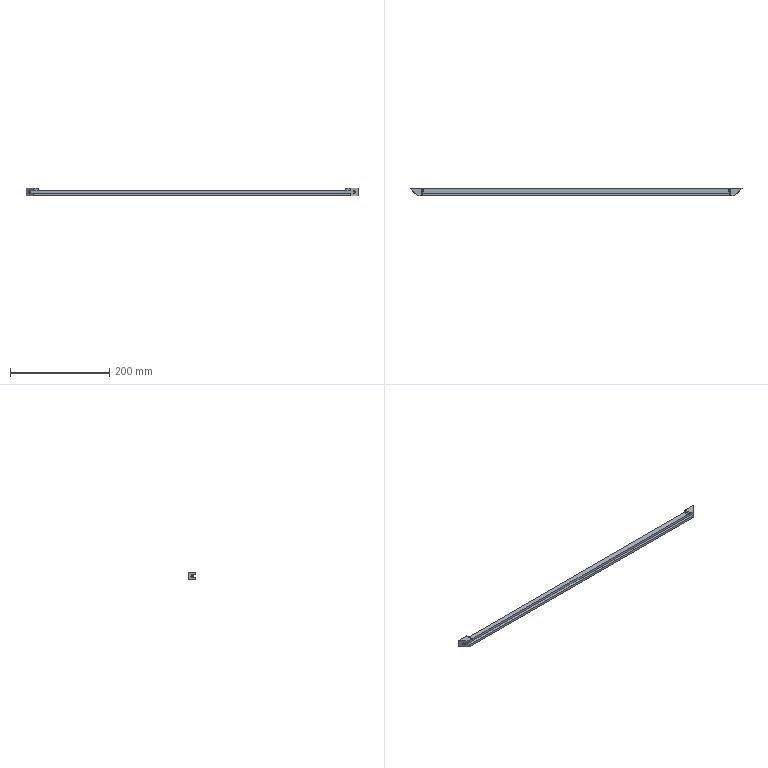Component | SolidWorks | AUTO-SpinDryWashing-01-03000006-1 | 1 solid | 30 faces | box 670 x 15 x 15 mm | volume 84011 mm3 | plane 18 | cylinder 12 | commonest cylinder face diameters 4.5 x4 8 x4 4 x4 | material AISI 304
STEP:
#1=CARTESIAN_POINT('',(-12.973,31.202,2.264));
#2=VERTEX_POINT('',#1);
#3=CARTESIAN_POINT('',(-12.848,31.076,2.264));
#4=VERTEX_POINT('',#3);
#5=CARTESIAN_POINT('',(-12.911,31.139,2.264));
#6=DIRECTION('',(-0.7071,-0.7071,-0.));
#7=DIRECTION('',(0.7071,-0.7071,0.));
#8=AXIS2_PLACEMENT_3D('',#5,#6,#7);
#9=CIRCLE('',#8,0.08858);
#10=EDGE_CURVE('',#2,#4,#9,.T.);
#11=ORIENTED_EDGE('',*,*,#10,.T.);
#12=CARTESIAN_POINT('',(-12.737,31.188,2.264));
#13=VERTEX_POINT('',#12);
#14=CARTESIAN_POINT('',(-12.458,31.466,2.264));
#15=DIRECTION('',(0.7071,0.7071,0.));
#16=VECTOR('',#15,39.37);
#17=LINE('',#14,#16);
#18=EDGE_CURVE('',#4,#13,#17,.T.);
#19=ORIENTED_EDGE('',*,*,#18,.T.);
#20=CARTESIAN_POINT('',(-12.862,31.313,2.264));
#21=VERTEX_POINT('',#20);
#22=CARTESIAN_POINT('',(-12.799,31.25,2.264));
#23=DIRECTION('',(0.7071,0.7071,0.));
#24=DIRECTION('',(-0.7071,0.7071,0.));
#25=AXIS2_PLACEMENT_3D('',#22,#23,#24);
#26=CIRCLE('',#25,0.08858);
#27=EDGE_CURVE('',#13,#21,#26,.T.);
#28=ORIENTED_EDGE('',*,*,#27,.T.);
#29=CARTESIAN_POINT('',(-12.583,31.591,2.264));
#30=DIRECTION('',(0.7071,0.7071,0.));
#31=VECTOR('',#30,39.37);
#32=LINE('',#29,#31);
#33=EDGE_CURVE('',#2,#21,#32,.T.);
#34=ORIENTED_EDGE('',*,*,#33,.F.);
#35=EDGE_LOOP('',(#11,#19,#28,#34));
#36=FACE_OUTER_BOUND('',#35,.T.);
#37=CARTESIAN_POINT('',(-12.521,31.529,2.264));
#38=DIRECTION('',(0.7071,0.7071,0.));
#39=DIRECTION('',(-0.7071,0.7071,0.));
#40=AXIS2_PLACEMENT_3D('',#37,#38,#39);
#41=CYLINDRICAL_SURFACE('',#40,0.08858);
#42=ADVANCED_FACE('',(#36),#41,.F.);
#43=CARTESIAN_POINT('',(-12.688,31.139,2.264));
#44=VERTEX_POINT('',#43);
#45=CARTESIAN_POINT('',(-12.911,31.362,2.264));
#46=VERTEX_POINT('',#45);
#47=CARTESIAN_POINT('',(-12.799,31.25,2.264));
#48=DIRECTION('',(0.7071,0.7071,0.));
#49=DIRECTION('',(-0.7071,0.7071,0.));
#50=AXIS2_PLACEMENT_3D('',#47,#48,#49);
#51=CIRCLE('',#50,0.1575);
#52=EDGE_CURVE('',#44,#46,#51,.T.);
#53=ORIENTED_EDGE('',*,*,#52,.F.);
#54=CARTESIAN_POINT('',(-12.409,31.417,2.264));
#55=VERTEX_POINT('',#54);
#56=CARTESIAN_POINT('',(-12.409,31.417,2.264));
#57=DIRECTION('',(0.7071,0.7071,0.));
#58=VECTOR('',#57,39.37);
#59=LINE('',#56,#58);
#60=EDGE_CURVE('',#44,#55,#59,.T.);
#61=ORIENTED_EDGE('',*,*,#60,.T.);
#62=CARTESIAN_POINT('',(-12.855,31.417,2.264));
#63=VERTEX_POINT('',#62);
#64=CARTESIAN_POINT('',(-12.855,31.417,2.264));
#65=CARTESIAN_POINT('',(-12.855,31.417,1.949));
#66=CARTESIAN_POINT('',(-12.409,31.417,1.949));
#67=CARTESIAN_POINT('',(-12.409,31.417,2.264));
#68=(BOUNDED_CURVE()B_SPLINE_CURVE(3,(#64,#65,#66,#67),.UNSPECIFIED.,.F.,.T.)B_SPLINE_CURVE_WITH_KNOTS((4,4),(3.142,6.283),.UNSPECIFIED.)CURVE()GEOMETRIC_REPRESENTATION_ITEM()RATIONAL_B_SPLINE_CURVE((1.,0.3333,0.3333,1.))REPRESENTATION_ITEM(''));
#69=EDGE_CURVE('',#63,#55,#68,.T.);
#70=ORIENTED_EDGE('',*,*,#69,.F.);
#71=CARTESIAN_POINT('',(-12.632,31.64,2.264));
#72=DIRECTION('',(0.7071,0.7071,0.));
#73=VECTOR('',#72,39.37);
#74=LINE('',#71,#73);
#75=EDGE_CURVE('',#46,#63,#74,.T.);
#76=ORIENTED_EDGE('',*,*,#75,.F.);
#77=EDGE_LOOP('',(#53,#61,#70,#76));
#78=FACE_OUTER_BOUND('',#77,.T.);
#79=CARTESIAN_POINT('',(-12.521,31.529,2.264));
#80=DIRECTION('',(0.7071,0.7071,0.));
#81=DIRECTION('',(-0.7071,0.7071,0.));
#82=AXIS2_PLACEMENT_3D('',#79,#80,#81);
#83=CYLINDRICAL_SURFACE('',#82,0.1575);
#84=ADVANCED_FACE('',(#78),#83,.F.);
#85=CARTESIAN_POINT('',(12.973,31.202,2.264));
#86=VERTEX_POINT('',#85);
#87=CARTESIAN_POINT('',(12.848,31.076,2.264));
#88=VERTEX_POINT('',#87);
#89=CARTESIAN_POINT('',(12.911,31.139,2.264));
#90=DIRECTION('',(-0.7071,0.7071,-0.));
#91=DIRECTION('',(-0.7071,-0.7071,0.));
#92=AXIS2_PLACEMENT_3D('',#89,#90,#91);
#93=CIRCLE('',#92,0.08858);
#94=EDGE_CURVE('',#86,#88,#93,.T.);
#95=ORIENTED_EDGE('',*,*,#94,.F.);
#96=CARTESIAN_POINT('',(12.862,31.313,2.264));
#97=VERTEX_POINT('',#96);
#98=CARTESIAN_POINT('',(12.583,31.591,2.264));
#99=DIRECTION('',(-0.7071,0.7071,-0.));
#100=VECTOR('',#99,39.37);
#101=LINE('',#98,#100);
#102=EDGE_CURVE('',#86,#97,#101,.T.);
#103=ORIENTED_EDGE('',*,*,#102,.T.);
#104=CARTESIAN_POINT('',(12.737,31.188,2.264));
#105=VERTEX_POINT('',#104);
#106=CARTESIAN_POINT('',(12.799,31.25,2.264));
#107=DIRECTION('',(-0.7071,0.7071,-0.));
#108=DIRECTION('',(-0.7071,-0.7071,0.));
#109=AXIS2_PLACEMENT_3D('',#106,#107,#108);
#110=CIRCLE('',#109,0.08858);
#111=EDGE_CURVE('',#97,#105,#110,.T.);
#112=ORIENTED_EDGE('',*,*,#111,.T.);
#113=CARTESIAN_POINT('',(12.458,31.466,2.264));
#114=DIRECTION('',(-0.7071,0.7071,-0.));
#115=VECTOR('',#114,39.37);
#116=LINE('',#113,#115);
#117=EDGE_CURVE('',#88,#105,#116,.T.);
#118=ORIENTED_EDGE('',*,*,#117,.F.);
#119=EDGE_LOOP('',(#95,#103,#112,#118));
#120=FACE_OUTER_BOUND('',#119,.T.);
#121=CARTESIAN_POINT('',(12.521,31.529,2.264));
#122=DIRECTION('',(-0.7071,0.7071,-0.));
#123=DIRECTION('',(-0.7071,-0.7071,0.));
#124=AXIS2_PLACEMENT_3D('',#121,#122,#123);
#125=CYLINDRICAL_SURFACE('',#124,0.08858);
#126=ADVANCED_FACE('',(#120),#125,.F.);
#127=CARTESIAN_POINT('',(12.911,31.362,2.264));
#128=VERTEX_POINT('',#127);
#129=CARTESIAN_POINT('',(12.688,31.139,2.264));
#130=VERTEX_POINT('',#129);
#131=CARTESIAN_POINT('',(12.799,31.25,2.264));
#132=DIRECTION('',(-0.7071,0.7071,-0.));
#133=DIRECTION('',(-0.7071,-0.7071,0.));
#134=AXIS2_PLACEMENT_3D('',#131,#132,#133);
#135=CIRCLE('',#134,0.1575);
#136=EDGE_CURVE('',#128,#130,#135,.T.);
#137=ORIENTED_EDGE('',*,*,#136,.F.);
#138=CARTESIAN_POINT('',(12.855,31.417,2.264));
#139=VERTEX_POINT('',#138);
#140=CARTESIAN_POINT('',(12.632,31.64,2.264));
#141=DIRECTION('',(-0.7071,0.7071,-0.));
#142=VECTOR('',#141,39.37);
#143=LINE('',#140,#142);
#144=EDGE_CURVE('',#128,#139,#143,.T.);
#145=ORIENTED_EDGE('',*,*,#144,.T.);
#146=CARTESIAN_POINT('',(12.409,31.417,2.264));
#147=VERTEX_POINT('',#146);
#148=CARTESIAN_POINT('',(12.409,31.417,2.264));
#149=CARTESIAN_POINT('',(12.409,31.417,1.949));
#150=CARTESIAN_POINT('',(12.855,31.417,1.949));
#151=CARTESIAN_POINT('',(12.855,31.417,2.264));
#152=(BOUNDED_CURVE()B_SPLINE_CURVE(3,(#148,#149,#150,#151),.UNSPECIFIED.,.F.,.F.)B_SPLINE_CURVE_WITH_KNOTS((4,4),(-0.,3.142),.UNSPECIFIED.)CURVE()GEOMETRIC_REPRESENTATION_ITEM()RATIONAL_B_SPLINE_CURVE((1.,0.3333,0.3333,1.))REPRESENTATION_ITEM(''));
#153=EDGE_CURVE('',#147,#139,#152,.T.);
#154=ORIENTED_EDGE('',*,*,#153,.F.);
#155=CARTESIAN_POINT('',(12.409,31.417,2.264));
#156=DIRECTION('',(-0.7071,0.7071,-0.));
#157=VECTOR('',#156,39.37);
#158=LINE('',#155,#157);
#159=EDGE_CURVE('',#130,#147,#158,.T.);
#160=ORIENTED_EDGE('',*,*,#159,.F.);
#161=EDGE_LOOP('',(#137,#145,#154,#160));
#162=FACE_OUTER_BOUND('',#161,.T.);
#163=CARTESIAN_POINT('',(12.521,31.529,2.264));
#164=DIRECTION('',(-0.7071,0.7071,-0.));
#165=DIRECTION('',(-0.7071,-0.7071,0.));
#166=AXIS2_PLACEMENT_3D('',#163,#164,#165);
#167=CYLINDRICAL_SURFACE('',#166,0.1575);
#168=ADVANCED_FACE('',(#162),#167,.F.);
#169=CARTESIAN_POINT('',(12.598,30.827,2.559));
#170=VERTEX_POINT('',#169);
#171=CARTESIAN_POINT('',(12.283,30.827,2.559));
#172=VERTEX_POINT('',#171);
#173=CARTESIAN_POINT('',(13.189,30.827,2.559));
#174=DIRECTION('',(-1.,0.,-0.));
#175=VECTOR('',#174,39.37);
#176=LINE('',#173,#175);
#177=EDGE_CURVE('',#170,#172,#176,.T.);
#178=ORIENTED_EDGE('',*,*,#177,.T.);
#179=CARTESIAN_POINT('',(12.205,30.827,2.48));
#180=VERTEX_POINT('',#179);
#181=CARTESIAN_POINT('',(12.283,30.827,2.48));
#182=DIRECTION('',(0.,-1.,0.));
#183=DIRECTION('',(1.,0.,0.));
#184=AXIS2_PLACEMENT_3D('',#181,#182,#183);
#185=CIRCLE('',#184,0.07874);
#186=EDGE_CURVE('',#172,#180,#185,.T.);
#187=ORIENTED_EDGE('',*,*,#186,.T.);
#188=CARTESIAN_POINT('',(12.205,30.827,2.362));
#189=VERTEX_POINT('',#188);
#190=CARTESIAN_POINT('',(12.205,30.827,1.969));
#191=DIRECTION('',(-0.,-0.,1.));
#192=VECTOR('',#191,39.37);
#193=LINE('',#190,#192);
#194=EDGE_CURVE('',#189,#180,#193,.T.);
#195=ORIENTED_EDGE('',*,*,#194,.F.);
#196=CARTESIAN_POINT('',(12.598,30.827,2.362));
#197=VERTEX_POINT('',#196);
#198=CARTESIAN_POINT('',(13.189,30.827,2.362));
#199=DIRECTION('',(-1.,0.,-0.));
#200=VECTOR('',#199,39.37);
#201=LINE('',#198,#200);
#202=EDGE_CURVE('',#197,#189,#201,.T.);
#203=ORIENTED_EDGE('',*,*,#202,.F.);
#204=CARTESIAN_POINT('',(12.598,30.827,1.969));
#205=DIRECTION('',(-0.,-0.,1.));
#206=VECTOR('',#205,39.37);
#207=LINE('',#204,#206);
#208=EDGE_CURVE('',#197,#170,#207,.T.);
#209=ORIENTED_EDGE('',*,*,#208,.T.);
#210=EDGE_LOOP('',(#178,#187,#195,#203,#209));
#211=FACE_OUTER_BOUND('',#210,.T.);
#212=CARTESIAN_POINT('',(13.189,30.827,1.969));
#213=DIRECTION('',(-0.,-1.,0.));
#214=DIRECTION('',(1.,-0.,0.));
#215=AXIS2_PLACEMENT_3D('',#212,#213,#214);
#216=PLANE('',#215);
#217=ADVANCED_FACE('',(#211),#216,.T.);
#218=ORIENTED_EDGE('',*,*,#202,.T.);
#219=CARTESIAN_POINT('',(12.205,31.024,2.362));
#220=VERTEX_POINT('',#219);
#221=CARTESIAN_POINT('',(12.205,27.599,2.362));
#222=DIRECTION('',(0.,1.,-0.));
#223=VECTOR('',#222,39.37);
#224=LINE('',#221,#223);
#225=EDGE_CURVE('',#189,#220,#224,.T.);
#226=ORIENTED_EDGE('',*,*,#225,.T.);
#227=CARTESIAN_POINT('',(12.795,31.024,2.362));
#228=VERTEX_POINT('',#227);
#229=CARTESIAN_POINT('',(13.189,31.024,2.362));
#230=DIRECTION('',(-1.,0.,-0.));
#231=VECTOR('',#230,39.37);
#232=LINE('',#229,#231);
#233=EDGE_CURVE('',#228,#220,#232,.T.);
#234=ORIENTED_EDGE('',*,*,#233,.F.);
#235=CARTESIAN_POINT('',(13.189,31.417,2.362));
#236=DIRECTION('',(-0.7071,-0.7071,-0.));
#237=VECTOR('',#236,39.37);
#238=LINE('',#235,#237);
#239=EDGE_CURVE('',#228,#197,#238,.T.);
#240=ORIENTED_EDGE('',*,*,#239,.T.);
#241=EDGE_LOOP('',(#218,#226,#234,#240));
#242=FACE_OUTER_BOUND('',#241,.T.);
#243=CARTESIAN_POINT('',(13.189,31.417,2.362));
#244=DIRECTION('',(-0.,-0.,1.));
#245=DIRECTION('',(-1.,0.,-0.));
#246=AXIS2_PLACEMENT_3D('',#243,#244,#245);
#247=PLANE('',#246);
#248=ADVANCED_FACE('',(#242),#247,.F.);
#249=CARTESIAN_POINT('',(13.189,31.417,2.559));
#250=VERTEX_POINT('',#249);
#251=CARTESIAN_POINT('',(12.283,31.417,2.559));
#252=VERTEX_POINT('',#251);
#253=CARTESIAN_POINT('',(13.189,31.417,2.559));
#254=DIRECTION('',(-1.,0.,-0.));
#255=VECTOR('',#254,39.37);
#256=LINE('',#253,#255);
#257=EDGE_CURVE('',#250,#252,#256,.T.);
#258=ORIENTED_EDGE('',*,*,#257,.T.);
#259=CARTESIAN_POINT('',(12.283,31.417,2.559));
#260=DIRECTION('',(0.,-1.,0.));
#261=VECTOR('',#260,39.37);
#262=LINE('',#259,#261);
#263=EDGE_CURVE('',#252,#172,#262,.T.);
#264=ORIENTED_EDGE('',*,*,#263,.T.);
#265=ORIENTED_EDGE('',*,*,#177,.F.);
#266=CARTESIAN_POINT('',(13.189,31.417,2.559));
#267=DIRECTION('',(-0.7071,-0.7071,-0.));
#268=VECTOR('',#267,39.37);
#269=LINE('',#266,#268);
#270=EDGE_CURVE('',#250,#170,#269,.T.);
#271=ORIENTED_EDGE('',*,*,#270,.F.);
#272=EDGE_LOOP('',(#258,#264,#265,#271));
#273=FACE_OUTER_BOUND('',#272,.T.);
#274=CARTESIAN_POINT('',(13.189,31.417,2.559));
#275=DIRECTION('',(0.,0.,-1.));
#276=DIRECTION('',(1.,-0.,0.));
#277=AXIS2_PLACEMENT_3D('',#274,#275,#276);
#278=PLANE('',#277);
#279=ADVANCED_FACE('',(#273),#278,.F.);
#280=CARTESIAN_POINT('',(-12.205,30.827,2.48));
#281=VERTEX_POINT('',#280);
#282=CARTESIAN_POINT('',(-12.205,30.827,2.362));
#283=VERTEX_POINT('',#282);
#284=CARTESIAN_POINT('',(-12.205,30.827,1.969));
#285=DIRECTION('',(0.,0.,-1.));
#286=VECTOR('',#285,39.37);
#287=LINE('',#284,#286);
#288=EDGE_CURVE('',#281,#283,#287,.T.);
#289=ORIENTED_EDGE('',*,*,#288,.F.);
#290=CARTESIAN_POINT('',(-12.283,30.827,2.559));
#291=VERTEX_POINT('',#290);
#292=CARTESIAN_POINT('',(-12.283,30.827,2.48));
#293=DIRECTION('',(0.,-1.,0.));
#294=DIRECTION('',(1.,0.,0.));
#295=AXIS2_PLACEMENT_3D('',#292,#293,#294);
#296=CIRCLE('',#295,0.07874);
#297=EDGE_CURVE('',#281,#291,#296,.T.);
#298=ORIENTED_EDGE('',*,*,#297,.T.);
#299=CARTESIAN_POINT('',(-12.598,30.827,2.559));
#300=VERTEX_POINT('',#299);
#301=CARTESIAN_POINT('',(13.189,30.827,2.559));
#302=DIRECTION('',(-1.,0.,-0.));
#303=VECTOR('',#302,39.37);
#304=LINE('',#301,#303);
#305=EDGE_CURVE('',#291,#300,#304,.T.);
#306=ORIENTED_EDGE('',*,*,#305,.T.);
#307=CARTESIAN_POINT('',(-12.598,30.827,2.362));
#308=VERTEX_POINT('',#307);
#309=CARTESIAN_POINT('',(-12.598,30.827,1.969));
#310=DIRECTION('',(-0.,-0.,1.));
#311=VECTOR('',#310,39.37);
#312=LINE('',#309,#311);
#313=EDGE_CURVE('',#308,#300,#312,.T.);
#314=ORIENTED_EDGE('',*,*,#313,.F.);
#315=CARTESIAN_POINT('',(13.189,30.827,2.362));
#316=DIRECTION('',(-1.,0.,-0.));
#317=VECTOR('',#316,39.37);
#318=LINE('',#315,#317);
#319=EDGE_CURVE('',#283,#308,#318,.T.);
#320=ORIENTED_EDGE('',*,*,#319,.F.);
#321=EDGE_LOOP('',(#289,#298,#306,#314,#320));
#322=FACE_OUTER_BOUND('',#321,.T.);
#323=CARTESIAN_POINT('',(13.189,30.827,1.969));
#324=DIRECTION('',(-0.,-1.,0.));
#325=DIRECTION('',(1.,-0.,0.));
#326=AXIS2_PLACEMENT_3D('',#323,#324,#325);
#327=PLANE('',#326);
#328=ADVANCED_FACE('',(#322),#327,.T.);
#329=CARTESIAN_POINT('',(-12.205,31.024,2.362));
#330=VERTEX_POINT('',#329);
#331=CARTESIAN_POINT('',(-12.795,31.024,2.362));
#332=VERTEX_POINT('',#331);
#333=CARTESIAN_POINT('',(13.189,31.024,2.362));
#334=DIRECTION('',(-1.,0.,-0.));
#335=VECTOR('',#334,39.37);
#336=LINE('',#333,#335);
#337=EDGE_CURVE('',#330,#332,#336,.T.);
#338=ORIENTED_EDGE('',*,*,#337,.F.);
#339=CARTESIAN_POINT('',(-12.205,27.599,2.362));
#340=DIRECTION('',(-0.,-1.,0.));
#341=VECTOR('',#340,39.37);
#342=LINE('',#339,#341);
#343=EDGE_CURVE('',#330,#283,#342,.T.);
#344=ORIENTED_EDGE('',*,*,#343,.T.);
#345=ORIENTED_EDGE('',*,*,#319,.T.);
#346=CARTESIAN_POINT('',(0.,18.228,2.362));
#347=DIRECTION('',(0.7071,-0.7071,0.));
#348=VECTOR('',#347,39.37);
#349=LINE('',#346,#348);
#350=EDGE_CURVE('',#332,#308,#349,.T.);
#351=ORIENTED_EDGE('',*,*,#350,.F.);
#352=EDGE_LOOP('',(#338,#344,#345,#351));
#353=FACE_OUTER_BOUND('',#352,.T.);
#354=CARTESIAN_POINT('',(13.189,31.417,2.362));
#355=DIRECTION('',(-0.,-0.,1.));
#356=DIRECTION('',(-1.,0.,-0.));
#357=AXIS2_PLACEMENT_3D('',#354,#355,#356);
#358=PLANE('',#357);
#359=ADVANCED_FACE('',(#353),#358,.F.);
#360=ORIENTED_EDGE('',*,*,#233,.T.);
#361=CARTESIAN_POINT('',(12.205,31.024,2.441));
#362=VERTEX_POINT('',#361);
#363=CARTESIAN_POINT('',(12.205,31.024,2.362));
#364=DIRECTION('',(-0.,-0.,-1.));
#365=VECTOR('',#364,39.37);
#366=LINE('',#363,#365);
#367=EDGE_CURVE('',#362,#220,#366,.T.);
#368=ORIENTED_EDGE('',*,*,#367,.F.);
#369=CARTESIAN_POINT('',(12.126,31.024,2.362));
#370=VERTEX_POINT('',#369);
#371=CARTESIAN_POINT('',(12.126,31.024,2.441));
#372=DIRECTION('',(-0.,1.,-0.));
#373=DIRECTION('',(0.,0.,-1.));
#374=AXIS2_PLACEMENT_3D('',#371,#372,#373);
#375=CIRCLE('',#374,0.07874);
#376=EDGE_CURVE('',#362,#370,#375,.T.);
#377=ORIENTED_EDGE('',*,*,#376,.T.);
#378=CARTESIAN_POINT('',(-12.126,31.024,2.362));
#379=VERTEX_POINT('',#378);
#380=CARTESIAN_POINT('',(13.189,31.024,2.362));
#381=DIRECTION('',(-1.,0.,-0.));
#382=VECTOR('',#381,39.37);
#383=LINE('',#380,#382);
#384=EDGE_CURVE('',#370,#379,#383,.T.);
#385=ORIENTED_EDGE('',*,*,#384,.T.);
#386=CARTESIAN_POINT('',(-12.205,31.024,2.441));
#387=VERTEX_POINT('',#386);
#388=CARTESIAN_POINT('',(-12.126,31.024,2.441));
#389=DIRECTION('',(-0.,1.,-0.));
#390=DIRECTION('',(0.,0.,-1.));
#391=AXIS2_PLACEMENT_3D('',#388,#389,#390);
#392=CIRCLE('',#391,0.07874);
#393=EDGE_CURVE('',#379,#387,#392,.T.);
#394=ORIENTED_EDGE('',*,*,#393,.T.);
#395=CARTESIAN_POINT('',(-12.205,31.024,2.362));
#396=DIRECTION('',(0.,0.,1.));
#397=VECTOR('',#396,39.37);
#398=LINE('',#395,#397);
#399=EDGE_CURVE('',#330,#387,#398,.T.);
#400=ORIENTED_EDGE('',*,*,#399,.F.);
#401=ORIENTED_EDGE('',*,*,#337,.T.);
#402=CARTESIAN_POINT('',(-12.795,31.024,2.165));
#403=VERTEX_POINT('',#402);
#404=CARTESIAN_POINT('',(-12.795,31.024,1.969));
#405=DIRECTION('',(0.,-0.,-1.));
#406=VECTOR('',#405,39.37);
#407=LINE('',#404,#406);
#408=EDGE_CURVE('',#332,#403,#407,.T.);
#409=ORIENTED_EDGE('',*,*,#408,.T.);
#410=CARTESIAN_POINT('',(12.795,31.024,2.165));
#411=VERTEX_POINT('',#410);
#412=CARTESIAN_POINT('',(13.189,31.024,2.165));
#413=DIRECTION('',(-1.,0.,-0.));
#414=VECTOR('',#413,39.37);
#415=LINE('',#412,#414);
#416=EDGE_CURVE('',#411,#403,#415,.T.);
#417=ORIENTED_EDGE('',*,*,#416,.F.);
#418=CARTESIAN_POINT('',(12.795,31.024,1.969));
#419=DIRECTION('',(-0.,-0.,-1.));
#420=VECTOR('',#419,39.37);
#421=LINE('',#418,#420);
#422=EDGE_CURVE('',#228,#411,#421,.T.);
#423=ORIENTED_EDGE('',*,*,#422,.F.);
#424=EDGE_LOOP('',(#360,#368,#377,#385,#394,#400,#401,#409,#417,#423));
#425=FACE_OUTER_BOUND('',#424,.T.);
#426=CARTESIAN_POINT('',(13.189,31.024,1.969));
#427=DIRECTION('',(0.,-1.,0.));
#428=DIRECTION('',(-0.,-0.,-1.));
#429=AXIS2_PLACEMENT_3D('',#426,#427,#428);
#430=PLANE('',#429);
#431=ADVANCED_FACE('',(#425),#430,.T.);
#432=ORIENTED_EDGE('',*,*,#416,.T.);
#433=CARTESIAN_POINT('',(-12.598,30.827,2.165));
#434=VERTEX_POINT('',#433);
#435=CARTESIAN_POINT('',(0.,18.228,2.165));
#436=DIRECTION('',(0.7071,-0.7071,0.));
#437=VECTOR('',#436,39.37);
#438=LINE('',#435,#437);
#439=EDGE_CURVE('',#403,#434,#438,.T.);
#440=ORIENTED_EDGE('',*,*,#439,.T.);
#441=CARTESIAN_POINT('',(12.598,30.827,2.165));
#442=VERTEX_POINT('',#441);
#443=CARTESIAN_POINT('',(13.189,30.827,2.165));
#444=DIRECTION('',(-1.,0.,-0.));
#445=VECTOR('',#444,39.37);
#446=LINE('',#443,#445);
#447=EDGE_CURVE('',#442,#434,#446,.T.);
#448=ORIENTED_EDGE('',*,*,#447,.F.);
#449=CARTESIAN_POINT('',(13.189,31.417,2.165));
#450=DIRECTION('',(-0.7071,-0.7071,-0.));
#451=VECTOR('',#450,39.37);
#452=LINE('',#449,#451);
#453=EDGE_CURVE('',#411,#442,#452,.T.);
#454=ORIENTED_EDGE('',*,*,#453,.F.);
#455=EDGE_LOOP('',(#432,#440,#448,#454));
#456=FACE_OUTER_BOUND('',#455,.T.);
#457=CARTESIAN_POINT('',(13.189,31.417,2.165));
#458=DIRECTION('',(-0.,-0.,1.));
#459=DIRECTION('',(0.,-1.,-0.));
#460=AXIS2_PLACEMENT_3D('',#457,#458,#459);
#461=PLANE('',#460);
#462=ADVANCED_FACE('',(#456),#461,.T.);
#463=ORIENTED_EDGE('',*,*,#447,.T.);
#464=CARTESIAN_POINT('',(-12.598,30.827,1.969));
#465=VERTEX_POINT('',#464);
#466=CARTESIAN_POINT('',(-12.598,30.827,1.969));
#467=DIRECTION('',(-0.,-0.,1.));
#468=VECTOR('',#467,39.37);
#469=LINE('',#466,#468);
#470=EDGE_CURVE('',#465,#434,#469,.T.);
#471=ORIENTED_EDGE('',*,*,#470,.F.);
#472=CARTESIAN_POINT('',(12.598,30.827,1.969));
#473=VERTEX_POINT('',#472);
#474=CARTESIAN_POINT('',(13.189,30.827,1.969));
#475=DIRECTION('',(-1.,0.,-0.));
#476=VECTOR('',#475,39.37);
#477=LINE('',#474,#476);
#478=EDGE_CURVE('',#473,#465,#477,.T.);
#479=ORIENTED_EDGE('',*,*,#478,.F.);
#480=CARTESIAN_POINT('',(12.598,30.827,1.969));
#481=DIRECTION('',(-0.,-0.,1.));
#482=VECTOR('',#481,39.37);
#483=LINE('',#480,#482);
#484=EDGE_CURVE('',#473,#442,#483,.T.);
#485=ORIENTED_EDGE('',*,*,#484,.T.);
#486=EDGE_LOOP('',(#463,#471,#479,#485));
#487=FACE_OUTER_BOUND('',#486,.T.);
#488=CARTESIAN_POINT('',(13.189,30.827,1.969));
#489=DIRECTION('',(-0.,-1.,0.));
#490=DIRECTION('',(1.,-0.,0.));
#491=AXIS2_PLACEMENT_3D('',#488,#489,#490);
#492=PLANE('',#491);
#493=ADVANCED_FACE('',(#487),#492,.T.);
#494=ORIENTED_EDGE('',*,*,#478,.T.);
#495=CARTESIAN_POINT('',(-13.189,31.417,1.969));
#496=VERTEX_POINT('',#495);
#497=CARTESIAN_POINT('',(-13.189,31.417,1.969));
#498=DIRECTION('',(0.7071,-0.7071,0.));
#499=VECTOR('',#498,39.37);
#500=LINE('',#497,#499);
#501=EDGE_CURVE('',#496,#465,#500,.T.);
#502=ORIENTED_EDGE('',*,*,#501,.F.);
#503=CARTESIAN_POINT('',(13.189,31.417,1.969));
#504=VERTEX_POINT('',#503);
#505=CARTESIAN_POINT('',(13.189,31.417,1.969));
#506=DIRECTION('',(-1.,0.,-0.));
#507=VECTOR('',#506,39.37);
#508=LINE('',#505,#507);
#509=EDGE_CURVE('',#504,#496,#508,.T.);
#510=ORIENTED_EDGE('',*,*,#509,.F.);
#511=CARTESIAN_POINT('',(13.189,31.417,1.969));
#512=DIRECTION('',(-0.7071,-0.7071,-0.));
#513=VECTOR('',#512,39.37);
#514=LINE('',#511,#513);
#515=EDGE_CURVE('',#504,#473,#514,.T.);
#516=ORIENTED_EDGE('',*,*,#515,.T.);
#517=EDGE_LOOP('',(#494,#502,#510,#516));
#518=FACE_OUTER_BOUND('',#517,.T.);
#519=CARTESIAN_POINT('',(13.189,31.417,1.969));
#520=DIRECTION('',(0.,0.,-1.));
#521=DIRECTION('',(1.,-0.,0.));
#522=AXIS2_PLACEMENT_3D('',#519,#520,#521);
#523=PLANE('',#522);
#524=ADVANCED_FACE('',(#518),#523,.T.);
#525=ORIENTED_EDGE('',*,*,#305,.F.);
#526=CARTESIAN_POINT('',(-12.283,31.417,2.559));
#527=VERTEX_POINT('',#526);
#528=CARTESIAN_POINT('',(-12.283,31.417,2.559));
#529=DIRECTION('',(-0.,1.,-0.));
#530=VECTOR('',#529,39.37);
#531=LINE('',#528,#530);
#532=EDGE_CURVE('',#291,#527,#531,.T.);
#533=ORIENTED_EDGE('',*,*,#532,.T.);
#534=CARTESIAN_POINT('',(-13.189,31.417,2.559));
#535=VERTEX_POINT('',#534);
#536=CARTESIAN_POINT('',(13.189,31.417,2.559));
#537=DIRECTION('',(-1.,0.,-0.));
#538=VECTOR('',#537,39.37);
#539=LINE('',#536,#538);
#540=EDGE_CURVE('',#527,#535,#539,.T.);
#541=ORIENTED_EDGE('',*,*,#540,.T.);
#542=CARTESIAN_POINT('',(-13.189,31.417,2.559));
#543=DIRECTION('',(0.7071,-0.7071,0.));
#544=VECTOR('',#543,39.37);
#545=LINE('',#542,#544);
#546=EDGE_CURVE('',#535,#300,#545,.T.);
#547=ORIENTED_EDGE('',*,*,#546,.T.);
#548=EDGE_LOOP('',(#525,#533,#541,#547));
#549=FACE_OUTER_BOUND('',#548,.T.);
#550=CARTESIAN_POINT('',(13.189,31.417,2.559));
#551=DIRECTION('',(0.,0.,-1.));
#552=DIRECTION('',(1.,-0.,0.));
#553=AXIS2_PLACEMENT_3D('',#550,#551,#552);
#554=PLANE('',#553);
#555=ADVANCED_FACE('',(#549),#554,.F.);
#556=ORIENTED_EDGE('',*,*,#69,.T.);
#557=CARTESIAN_POINT('',(-12.409,31.417,2.264));
#558=CARTESIAN_POINT('',(-12.409,31.417,2.579));
#559=CARTESIAN_POINT('',(-12.855,31.417,2.579));
#560=CARTESIAN_POINT('',(-12.855,31.417,2.264));
#561=(BOUNDED_CURVE()B_SPLINE_CURVE(3,(#557,#558,#559,#560),.UNSPECIFIED.,.F.,.F.)B_SPLINE_CURVE_WITH_KNOTS((4,4),(0.,3.142),.UNSPECIFIED.)CURVE()GEOMETRIC_REPRESENTATION_ITEM()RATIONAL_B_SPLINE_CURVE((1.,0.3333,0.3333,1.))REPRESENTATION_ITEM(''));
#562=EDGE_CURVE('',#55,#63,#561,.T.);
#563=ORIENTED_EDGE('',*,*,#562,.T.);
#564=EDGE_LOOP('',(#556,#563));
#565=FACE_BOUND('',#564,.T.);
#566=ORIENTED_EDGE('',*,*,#153,.T.);
#567=CARTESIAN_POINT('',(12.855,31.417,2.264));
#568=CARTESIAN_POINT('',(12.855,31.417,2.579));
#569=CARTESIAN_POINT('',(12.409,31.417,2.579));
#570=CARTESIAN_POINT('',(12.409,31.417,2.264));
#571=(BOUNDED_CURVE()B_SPLINE_CURVE(3,(#567,#568,#569,#570),.UNSPECIFIED.,.F.,.F.)B_SPLINE_CURVE_WITH_KNOTS((4,4),(3.142,6.283),.UNSPECIFIED.)CURVE()GEOMETRIC_REPRESENTATION_ITEM()RATIONAL_B_SPLINE_CURVE((1.,0.3333,0.3333,1.))REPRESENTATION_ITEM(''));
#572=EDGE_CURVE('',#139,#147,#571,.T.);
#573=ORIENTED_EDGE('',*,*,#572,.T.);
#574=EDGE_LOOP('',(#566,#573));
#575=FACE_BOUND('',#574,.T.);
#576=CARTESIAN_POINT('',(12.205,31.417,2.441));
#577=VERTEX_POINT('',#576);
#578=CARTESIAN_POINT('',(12.205,31.417,2.48));
#579=VERTEX_POINT('',#578);
#580=CARTESIAN_POINT('',(12.205,31.417,2.362));
#581=DIRECTION('',(-0.,-0.,1.));
#582=VECTOR('',#581,39.37);
#583=LINE('',#580,#582);
#584=EDGE_CURVE('',#577,#579,#583,.T.);
#585=ORIENTED_EDGE('',*,*,#584,.T.);
#586=CARTESIAN_POINT('',(12.283,31.417,2.48));
#587=DIRECTION('',(-0.,1.,-0.));
#588=DIRECTION('',(1.,0.,0.));
#589=AXIS2_PLACEMENT_3D('',#586,#587,#588);
#590=CIRCLE('',#589,0.07874);
#591=EDGE_CURVE('',#579,#252,#590,.T.);
#592=ORIENTED_EDGE('',*,*,#591,.T.);
#593=ORIENTED_EDGE('',*,*,#257,.F.);
#594=CARTESIAN_POINT('',(13.189,31.417,1.969));
#595=DIRECTION('',(-0.,-0.,1.));
#596=VECTOR('',#595,39.37);
#597=LINE('',#594,#596);
#598=EDGE_CURVE('',#504,#250,#597,.T.);
#599=ORIENTED_EDGE('',*,*,#598,.F.);
#600=ORIENTED_EDGE('',*,*,#509,.T.);
#601=CARTESIAN_POINT('',(-13.189,31.417,1.969));
#602=DIRECTION('',(-0.,-0.,1.));
#603=VECTOR('',#602,39.37);
#604=LINE('',#601,#603);
#605=EDGE_CURVE('',#496,#535,#604,.T.);
#606=ORIENTED_EDGE('',*,*,#605,.T.);
#607=ORIENTED_EDGE('',*,*,#540,.F.);
#608=CARTESIAN_POINT('',(-12.205,31.417,2.48));
#609=VERTEX_POINT('',#608);
#610=CARTESIAN_POINT('',(-12.283,31.417,2.48));
#611=DIRECTION('',(-0.,1.,-0.));
#612=DIRECTION('',(1.,0.,0.));
#613=AXIS2_PLACEMENT_3D('',#610,#611,#612);
#614=CIRCLE('',#613,0.07874);
#615=EDGE_CURVE('',#527,#609,#614,.T.);
#616=ORIENTED_EDGE('',*,*,#615,.T.);
#617=CARTESIAN_POINT('',(-12.205,31.417,2.441));
#618=VERTEX_POINT('',#617);
#619=CARTESIAN_POINT('',(-12.205,31.417,2.362));
#620=DIRECTION('',(-0.,-0.,1.));
#621=VECTOR('',#620,39.37);
#622=LINE('',#619,#621);
#623=EDGE_CURVE('',#618,#609,#622,.T.);
#624=ORIENTED_EDGE('',*,*,#623,.F.);
#625=CARTESIAN_POINT('',(-12.126,31.417,2.362));
#626=VERTEX_POINT('',#625);
#627=CARTESIAN_POINT('',(-12.126,31.417,2.441));
#628=DIRECTION('',(0.,-1.,0.));
#629=DIRECTION('',(1.,0.,0.));
#630=AXIS2_PLACEMENT_3D('',#627,#628,#629);
#631=CIRCLE('',#630,0.07874);
#632=EDGE_CURVE('',#618,#626,#631,.T.);
#633=ORIENTED_EDGE('',*,*,#632,.T.);
#634=CARTESIAN_POINT('',(12.126,31.417,2.362));
#635=VERTEX_POINT('',#634);
#636=CARTESIAN_POINT('',(12.205,31.417,2.362));
#637=DIRECTION('',(-1.,0.,-0.));
#638=VECTOR('',#637,39.37);
#639=LINE('',#636,#638);
#640=EDGE_CURVE('',#635,#626,#639,.T.);
#641=ORIENTED_EDGE('',*,*,#640,.F.);
#642=CARTESIAN_POINT('',(12.126,31.417,2.441));
#643=DIRECTION('',(0.,-1.,0.));
#644=DIRECTION('',(1.,0.,0.));
#645=AXIS2_PLACEMENT_3D('',#642,#643,#644);
#646=CIRCLE('',#645,0.07874);
#647=EDGE_CURVE('',#635,#577,#646,.T.);
#648=ORIENTED_EDGE('',*,*,#647,.T.);
#649=EDGE_LOOP('',(#585,#592,#593,#599,#600,#606,#607,#616,#624,#633,#641,#648));
#650=FACE_OUTER_BOUND('',#649,.T.);
#651=CARTESIAN_POINT('',(13.189,31.417,1.969));
#652=DIRECTION('',(-0.,-1.,0.));
#653=DIRECTION('',(1.,-0.,0.));
#654=AXIS2_PLACEMENT_3D('',#651,#652,#653);
#655=PLANE('',#654);
#656=ADVANCED_FACE('',(#565,#575,#650),#655,.F.);
#657=CARTESIAN_POINT('',(12.911,31.139,2.264));
#658=DIRECTION('',(-0.7071,0.7071,-0.));
#659=DIRECTION('',(-0.7071,-0.7071,0.));
#660=AXIS2_PLACEMENT_3D('',#657,#658,#659);
#661=CIRCLE('',#660,0.08858);
#662=EDGE_CURVE('',#88,#86,#661,.T.);
#663=ORIENTED_EDGE('',*,*,#662,.T.);
#664=ORIENTED_EDGE('',*,*,#94,.T.);
#665=EDGE_LOOP('',(#663,#664));
#666=FACE_BOUND('',#665,.T.);
#667=ORIENTED_EDGE('',*,*,#422,.T.);
#668=ORIENTED_EDGE('',*,*,#453,.T.);
#669=ORIENTED_EDGE('',*,*,#484,.F.);
#670=ORIENTED_EDGE('',*,*,#515,.F.);
#671=ORIENTED_EDGE('',*,*,#598,.T.);
#672=ORIENTED_EDGE('',*,*,#270,.T.);
#673=ORIENTED_EDGE('',*,*,#208,.F.);
#674=ORIENTED_EDGE('',*,*,#239,.F.);
#675=EDGE_LOOP('',(#667,#668,#669,#670,#671,#672,#673,#674));
#676=FACE_OUTER_BOUND('',#675,.T.);
#677=CARTESIAN_POINT('',(13.189,31.417,1.969));
#678=DIRECTION('',(-0.7071,0.7071,-0.));
#679=DIRECTION('',(-0.7071,-0.7071,-0.));
#680=AXIS2_PLACEMENT_3D('',#677,#678,#679);
#681=PLANE('',#680);
#682=ADVANCED_FACE('',(#666,#676),#681,.F.);
#683=ORIENTED_EDGE('',*,*,#10,.F.);
#684=CARTESIAN_POINT('',(-12.911,31.139,2.264));
#685=DIRECTION('',(-0.7071,-0.7071,-0.));
#686=DIRECTION('',(0.7071,-0.7071,0.));
#687=AXIS2_PLACEMENT_3D('',#684,#685,#686);
#688=CIRCLE('',#687,0.08858);
#689=EDGE_CURVE('',#4,#2,#688,.T.);
#690=ORIENTED_EDGE('',*,*,#689,.F.);
#691=EDGE_LOOP('',(#683,#690));
#692=FACE_BOUND('',#691,.T.);
#693=ORIENTED_EDGE('',*,*,#350,.T.);
#694=ORIENTED_EDGE('',*,*,#313,.T.);
#695=ORIENTED_EDGE('',*,*,#546,.F.);
#696=ORIENTED_EDGE('',*,*,#605,.F.);
#697=ORIENTED_EDGE('',*,*,#501,.T.);
#698=ORIENTED_EDGE('',*,*,#470,.T.);
#699=ORIENTED_EDGE('',*,*,#439,.F.);
#700=ORIENTED_EDGE('',*,*,#408,.F.);
#701=EDGE_LOOP('',(#693,#694,#695,#696,#697,#698,#699,#700));
#702=FACE_OUTER_BOUND('',#701,.T.);
#703=CARTESIAN_POINT('',(-13.189,31.417,1.969));
#704=DIRECTION('',(-0.7071,-0.7071,-0.));
#705=DIRECTION('',(0.7071,-0.7071,0.));
#706=AXIS2_PLACEMENT_3D('',#703,#704,#705);
#707=PLANE('',#706);
#708=ADVANCED_FACE('',(#692,#702),#707,.T.);
#709=ORIENTED_EDGE('',*,*,#144,.F.);
#710=CARTESIAN_POINT('',(12.799,31.25,2.264));
#711=DIRECTION('',(-0.7071,0.7071,-0.));
#712=DIRECTION('',(-0.7071,-0.7071,0.));
#713=AXIS2_PLACEMENT_3D('',#710,#711,#712);
#714=CIRCLE('',#713,0.1575);
#715=EDGE_CURVE('',#130,#128,#714,.T.);
#716=ORIENTED_EDGE('',*,*,#715,.F.);
#717=ORIENTED_EDGE('',*,*,#159,.T.);
#718=ORIENTED_EDGE('',*,*,#572,.F.);
#719=EDGE_LOOP('',(#709,#716,#717,#718));
#720=FACE_OUTER_BOUND('',#719,.T.);
#721=CARTESIAN_POINT('',(12.521,31.529,2.264));
#722=DIRECTION('',(-0.7071,0.7071,-0.));
#723=DIRECTION('',(-0.7071,-0.7071,0.));
#724=AXIS2_PLACEMENT_3D('',#721,#722,#723);
#725=CYLINDRICAL_SURFACE('',#724,0.1575);
#726=ADVANCED_FACE('',(#720),#725,.F.);
#727=ORIENTED_EDGE('',*,*,#102,.F.);
#728=ORIENTED_EDGE('',*,*,#662,.F.);
#729=ORIENTED_EDGE('',*,*,#117,.T.);
#730=CARTESIAN_POINT('',(12.799,31.25,2.264));
#731=DIRECTION('',(-0.7071,0.7071,-0.));
#732=DIRECTION('',(-0.7071,-0.7071,0.));
#733=AXIS2_PLACEMENT_3D('',#730,#731,#732);
#734=CIRCLE('',#733,0.08858);
#735=EDGE_CURVE('',#105,#97,#734,.T.);
#736=ORIENTED_EDGE('',*,*,#735,.T.);
#737=EDGE_LOOP('',(#727,#728,#729,#736));
#738=FACE_OUTER_BOUND('',#737,.T.);
#739=CARTESIAN_POINT('',(12.521,31.529,2.264));
#740=DIRECTION('',(-0.7071,0.7071,-0.));
#741=DIRECTION('',(-0.7071,-0.7071,0.));
#742=AXIS2_PLACEMENT_3D('',#739,#740,#741);
#743=CYLINDRICAL_SURFACE('',#742,0.08858);
#744=ADVANCED_FACE('',(#738),#743,.F.);
#745=ORIENTED_EDGE('',*,*,#735,.F.);
#746=ORIENTED_EDGE('',*,*,#111,.F.);
#747=EDGE_LOOP('',(#745,#746));
#748=FACE_BOUND('',#747,.T.);
#749=ORIENTED_EDGE('',*,*,#715,.T.);
#750=ORIENTED_EDGE('',*,*,#136,.T.);
#751=EDGE_LOOP('',(#749,#750));
#752=FACE_OUTER_BOUND('',#751,.T.);
#753=CARTESIAN_POINT('',(12.799,31.25,2.352));
#754=DIRECTION('',(0.7071,-0.7071,0.));
#755=DIRECTION('',(0.7071,0.7071,0.));
#756=AXIS2_PLACEMENT_3D('',#753,#754,#755);
#757=PLANE('',#756);
#758=ADVANCED_FACE('',(#748,#752),#757,.F.);
#759=ORIENTED_EDGE('',*,*,#60,.F.);
#760=CARTESIAN_POINT('',(-12.799,31.25,2.264));
#761=DIRECTION('',(0.7071,0.7071,0.));
#762=DIRECTION('',(-0.7071,0.7071,0.));
#763=AXIS2_PLACEMENT_3D('',#760,#761,#762);
#764=CIRCLE('',#763,0.1575);
#765=EDGE_CURVE('',#46,#44,#764,.T.);
#766=ORIENTED_EDGE('',*,*,#765,.F.);
#767=ORIENTED_EDGE('',*,*,#75,.T.);
#768=ORIENTED_EDGE('',*,*,#562,.F.);
#769=EDGE_LOOP('',(#759,#766,#767,#768));
#770=FACE_OUTER_BOUND('',#769,.T.);
#771=CARTESIAN_POINT('',(-12.521,31.529,2.264));
#772=DIRECTION('',(0.7071,0.7071,0.));
#773=DIRECTION('',(-0.7071,0.7071,0.));
#774=AXIS2_PLACEMENT_3D('',#771,#772,#773);
#775=CYLINDRICAL_SURFACE('',#774,0.1575);
#776=ADVANCED_FACE('',(#770),#775,.F.);
#777=ORIENTED_EDGE('',*,*,#18,.F.);
#778=ORIENTED_EDGE('',*,*,#689,.T.);
#779=ORIENTED_EDGE('',*,*,#33,.T.);
#780=CARTESIAN_POINT('',(-12.799,31.25,2.264));
#781=DIRECTION('',(0.7071,0.7071,0.));
#782=DIRECTION('',(-0.7071,0.7071,0.));
#783=AXIS2_PLACEMENT_3D('',#780,#781,#782);
#784=CIRCLE('',#783,0.08858);
#785=EDGE_CURVE('',#21,#13,#784,.T.);
#786=ORIENTED_EDGE('',*,*,#785,.T.);
#787=EDGE_LOOP('',(#777,#778,#779,#786));
#788=FACE_OUTER_BOUND('',#787,.T.);
#789=CARTESIAN_POINT('',(-12.521,31.529,2.264));
#790=DIRECTION('',(0.7071,0.7071,0.));
#791=DIRECTION('',(-0.7071,0.7071,0.));
#792=AXIS2_PLACEMENT_3D('',#789,#790,#791);
#793=CYLINDRICAL_SURFACE('',#792,0.08858);
#794=ADVANCED_FACE('',(#788),#793,.F.);
#795=ORIENTED_EDGE('',*,*,#785,.F.);
#796=ORIENTED_EDGE('',*,*,#27,.F.);
#797=EDGE_LOOP('',(#795,#796));
#798=FACE_BOUND('',#797,.T.);
#799=ORIENTED_EDGE('',*,*,#765,.T.);
#800=ORIENTED_EDGE('',*,*,#52,.T.);
#801=EDGE_LOOP('',(#799,#800));
#802=FACE_OUTER_BOUND('',#801,.T.);
#803=CARTESIAN_POINT('',(-12.799,31.25,2.352));
#804=DIRECTION('',(-0.7071,-0.7071,-0.));
#805=DIRECTION('',(0.7071,-0.7071,0.));
#806=AXIS2_PLACEMENT_3D('',#803,#804,#805);
#807=PLANE('',#806);
#808=ADVANCED_FACE('',(#798,#802),#807,.F.);
#809=ORIENTED_EDGE('',*,*,#194,.T.);
#810=CARTESIAN_POINT('',(12.205,27.599,2.48));
#811=DIRECTION('',(-0.,1.,-0.));
#812=VECTOR('',#811,39.37);
#813=LINE('',#810,#812);
#814=EDGE_CURVE('',#180,#579,#813,.T.);
#815=ORIENTED_EDGE('',*,*,#814,.T.);
#816=ORIENTED_EDGE('',*,*,#584,.F.);
#817=CARTESIAN_POINT('',(12.205,27.599,2.441));
#818=DIRECTION('',(0.,-1.,0.));
#819=VECTOR('',#818,39.37);
#820=LINE('',#817,#819);
#821=EDGE_CURVE('',#577,#362,#820,.T.);
#822=ORIENTED_EDGE('',*,*,#821,.T.);
#823=ORIENTED_EDGE('',*,*,#367,.T.);
#824=ORIENTED_EDGE('',*,*,#225,.F.);
#825=EDGE_LOOP('',(#809,#815,#816,#822,#823,#824));
#826=FACE_OUTER_BOUND('',#825,.T.);
#827=CARTESIAN_POINT('',(12.205,27.599,2.362));
#828=DIRECTION('',(1.,-0.,0.));
#829=DIRECTION('',(-0.,-0.,1.));
#830=AXIS2_PLACEMENT_3D('',#827,#828,#829);
#831=PLANE('',#830);
#832=ADVANCED_FACE('',(#826),#831,.F.);
#833=ORIENTED_EDGE('',*,*,#623,.T.);
#834=CARTESIAN_POINT('',(-12.205,27.599,2.48));
#835=DIRECTION('',(0.,-1.,0.));
#836=VECTOR('',#835,39.37);
#837=LINE('',#834,#836);
#838=EDGE_CURVE('',#609,#281,#837,.T.);
#839=ORIENTED_EDGE('',*,*,#838,.T.);
#840=ORIENTED_EDGE('',*,*,#288,.T.);
#841=ORIENTED_EDGE('',*,*,#343,.F.);
#842=ORIENTED_EDGE('',*,*,#399,.T.);
#843=CARTESIAN_POINT('',(-12.205,27.599,2.441));
#844=DIRECTION('',(-0.,1.,-0.));
#845=VECTOR('',#844,39.37);
#846=LINE('',#843,#845);
#847=EDGE_CURVE('',#387,#618,#846,.T.);
#848=ORIENTED_EDGE('',*,*,#847,.T.);
#849=EDGE_LOOP('',(#833,#839,#840,#841,#842,#848));
#850=FACE_OUTER_BOUND('',#849,.T.);
#851=CARTESIAN_POINT('',(-12.205,27.599,2.362));
#852=DIRECTION('',(-1.,0.,-0.));
#853=DIRECTION('',(0.,0.,-1.));
#854=AXIS2_PLACEMENT_3D('',#851,#852,#853);
#855=PLANE('',#854);
#856=ADVANCED_FACE('',(#850),#855,.F.);
#857=ORIENTED_EDGE('',*,*,#640,.T.);
#858=CARTESIAN_POINT('',(-12.126,31.417,2.362));
#859=DIRECTION('',(0.,-1.,0.));
#860=VECTOR('',#859,39.37);
#861=LINE('',#858,#860);
#862=EDGE_CURVE('',#626,#379,#861,.T.);
#863=ORIENTED_EDGE('',*,*,#862,.T.);
#864=ORIENTED_EDGE('',*,*,#384,.F.);
#865=CARTESIAN_POINT('',(12.126,31.417,2.362));
#866=DIRECTION('',(-0.,1.,-0.));
#867=VECTOR('',#866,39.37);
#868=LINE('',#865,#867);
#869=EDGE_CURVE('',#370,#635,#868,.T.);
#870=ORIENTED_EDGE('',*,*,#869,.T.);
#871=EDGE_LOOP('',(#857,#863,#864,#870));
#872=FACE_OUTER_BOUND('',#871,.T.);
#873=CARTESIAN_POINT('',(0.,31.417,2.362));
#874=DIRECTION('',(-0.,-0.,1.));
#875=DIRECTION('',(-1.,0.,-0.));
#876=AXIS2_PLACEMENT_3D('',#873,#874,#875);
#877=PLANE('',#876);
#878=ADVANCED_FACE('',(#872),#877,.T.);
#879=ORIENTED_EDGE('',*,*,#186,.F.);
#880=ORIENTED_EDGE('',*,*,#263,.F.);
#881=ORIENTED_EDGE('',*,*,#591,.F.);
#882=ORIENTED_EDGE('',*,*,#814,.F.);
#883=EDGE_LOOP('',(#879,#880,#881,#882));
#884=FACE_OUTER_BOUND('',#883,.T.);
#885=CARTESIAN_POINT('',(12.283,27.599,2.48));
#886=DIRECTION('',(-0.,1.,-0.));
#887=DIRECTION('',(-1.,0.,0.));
#888=AXIS2_PLACEMENT_3D('',#885,#886,#887);
#889=CYLINDRICAL_SURFACE('',#888,0.07874);
#890=ADVANCED_FACE('',(#884),#889,.T.);
#891=ORIENTED_EDGE('',*,*,#615,.F.);
#892=ORIENTED_EDGE('',*,*,#532,.F.);
#893=ORIENTED_EDGE('',*,*,#297,.F.);
#894=ORIENTED_EDGE('',*,*,#838,.F.);
#895=EDGE_LOOP('',(#891,#892,#893,#894));
#896=FACE_OUTER_BOUND('',#895,.T.);
#897=CARTESIAN_POINT('',(-12.283,27.599,2.48));
#898=DIRECTION('',(0.,-1.,0.));
#899=DIRECTION('',(1.,0.,0.));
#900=AXIS2_PLACEMENT_3D('',#897,#898,#899);
#901=CYLINDRICAL_SURFACE('',#900,0.07874);
#902=ADVANCED_FACE('',(#896),#901,.T.);
#903=ORIENTED_EDGE('',*,*,#632,.F.);
#904=ORIENTED_EDGE('',*,*,#847,.F.);
#905=ORIENTED_EDGE('',*,*,#393,.F.);
#906=ORIENTED_EDGE('',*,*,#862,.F.);
#907=EDGE_LOOP('',(#903,#904,#905,#906));
#908=FACE_OUTER_BOUND('',#907,.T.);
#909=CARTESIAN_POINT('',(-12.126,31.417,2.441));
#910=DIRECTION('',(0.,-1.,0.));
#911=DIRECTION('',(1.,0.,0.));
#912=AXIS2_PLACEMENT_3D('',#909,#910,#911);
#913=CYLINDRICAL_SURFACE('',#912,0.07874);
#914=ADVANCED_FACE('',(#908),#913,.F.);
#915=ORIENTED_EDGE('',*,*,#376,.F.);
#916=ORIENTED_EDGE('',*,*,#821,.F.);
#917=ORIENTED_EDGE('',*,*,#647,.F.);
#918=ORIENTED_EDGE('',*,*,#869,.F.);
#919=EDGE_LOOP('',(#915,#916,#917,#918));
#920=FACE_OUTER_BOUND('',#919,.T.);
#921=CARTESIAN_POINT('',(12.126,31.417,2.441));
#922=DIRECTION('',(-0.,1.,-0.));
#923=DIRECTION('',(-1.,0.,0.));
#924=AXIS2_PLACEMENT_3D('',#921,#922,#923);
#925=CYLINDRICAL_SURFACE('',#924,0.07874);
#926=ADVANCED_FACE('',(#920),#925,.F.);
#927=CLOSED_SHELL('',(#42,#84,#126,#168,#217,#248,#279,#328,#359,#431,#462,#493,#524,#555,#656,#682,#708,#726,#744,#758,#776,#794,#808,#832,#856,#878,#890,#902,#914,#926));
#928=MANIFOLD_SOLID_BREP('',#927);
#929=CARTESIAN_POINT('',(0.,0.,0.));
#930=DIRECTION('',(0.,0.,1.));
#931=DIRECTION('',(1.,0.,0.));
#932=AXIS2_PLACEMENT_3D('',#929,#930,#931);
#933=(LENGTH_UNIT()NAMED_UNIT(*)SI_UNIT($,.METRE.));
#934=LENGTH_MEASURE_WITH_UNIT(LENGTH_MEASURE(0.0254),#933);
#935=DIMENSIONAL_EXPONENTS(1.,0.,0.,0.,0.,0.,0.);
#936=(CONVERSION_BASED_UNIT('',#934)LENGTH_UNIT()NAMED_UNIT(#935));
#937=UNCERTAINTY_MEASURE_WITH_UNIT(LENGTH_MEASURE(0.00001),#936,'','');
#938=(NAMED_UNIT(*)PLANE_ANGLE_UNIT()SI_UNIT($,.RADIAN.));
#939=(NAMED_UNIT(*)SI_UNIT($,.STERADIAN.)SOLID_ANGLE_UNIT());
#940=(GEOMETRIC_REPRESENTATION_CONTEXT(3)GLOBAL_UNCERTAINTY_ASSIGNED_CONTEXT((#937))GLOBAL_UNIT_ASSIGNED_CONTEXT((#936,#938,#939))REPRESENTATION_CONTEXT('',''));
#941=ADVANCED_BREP_SHAPE_REPRESENTATION('',(#928,#932),#940);
#942=COLOUR_RGB('',0.7922,0.8196,0.9333);
#943=FILL_AREA_STYLE_COLOUR('',#942);
#944=FILL_AREA_STYLE('',(#943));
#945=SURFACE_STYLE_FILL_AREA(#944);
#946=SURFACE_SIDE_STYLE('',(#945));
#947=SURFACE_STYLE_USAGE(.BOTH.,#946);
#948=PRESENTATION_STYLE_ASSIGNMENT((#947));
#949=STYLED_ITEM('',(#948),#928);
#950=(LENGTH_UNIT()NAMED_UNIT(*)SI_UNIT($,.METRE.));
#951=LENGTH_MEASURE_WITH_UNIT(LENGTH_MEASURE(0.0254),#950);
#952=DIMENSIONAL_EXPONENTS(1.,0.,0.,0.,0.,0.,0.);
#953=(CONVERSION_BASED_UNIT('',#951)LENGTH_UNIT()NAMED_UNIT(#952));
#954=UNCERTAINTY_MEASURE_WITH_UNIT(LENGTH_MEASURE(0.00001),#953,'','');
#955=(NAMED_UNIT(*)PLANE_ANGLE_UNIT()SI_UNIT($,.RADIAN.));
#956=(NAMED_UNIT(*)SI_UNIT($,.STERADIAN.)SOLID_ANGLE_UNIT());
#957=(GEOMETRIC_REPRESENTATION_CONTEXT(3)GLOBAL_UNCERTAINTY_ASSIGNED_CONTEXT((#954))GLOBAL_UNIT_ASSIGNED_CONTEXT((#953,#955,#956))REPRESENTATION_CONTEXT('',''));
#958=MECHANICAL_DESIGN_GEOMETRIC_PRESENTATION_REPRESENTATION('',(#949),#957);
#959=PRESENTATION_LAYER_ASSIGNMENT('','',(#949));